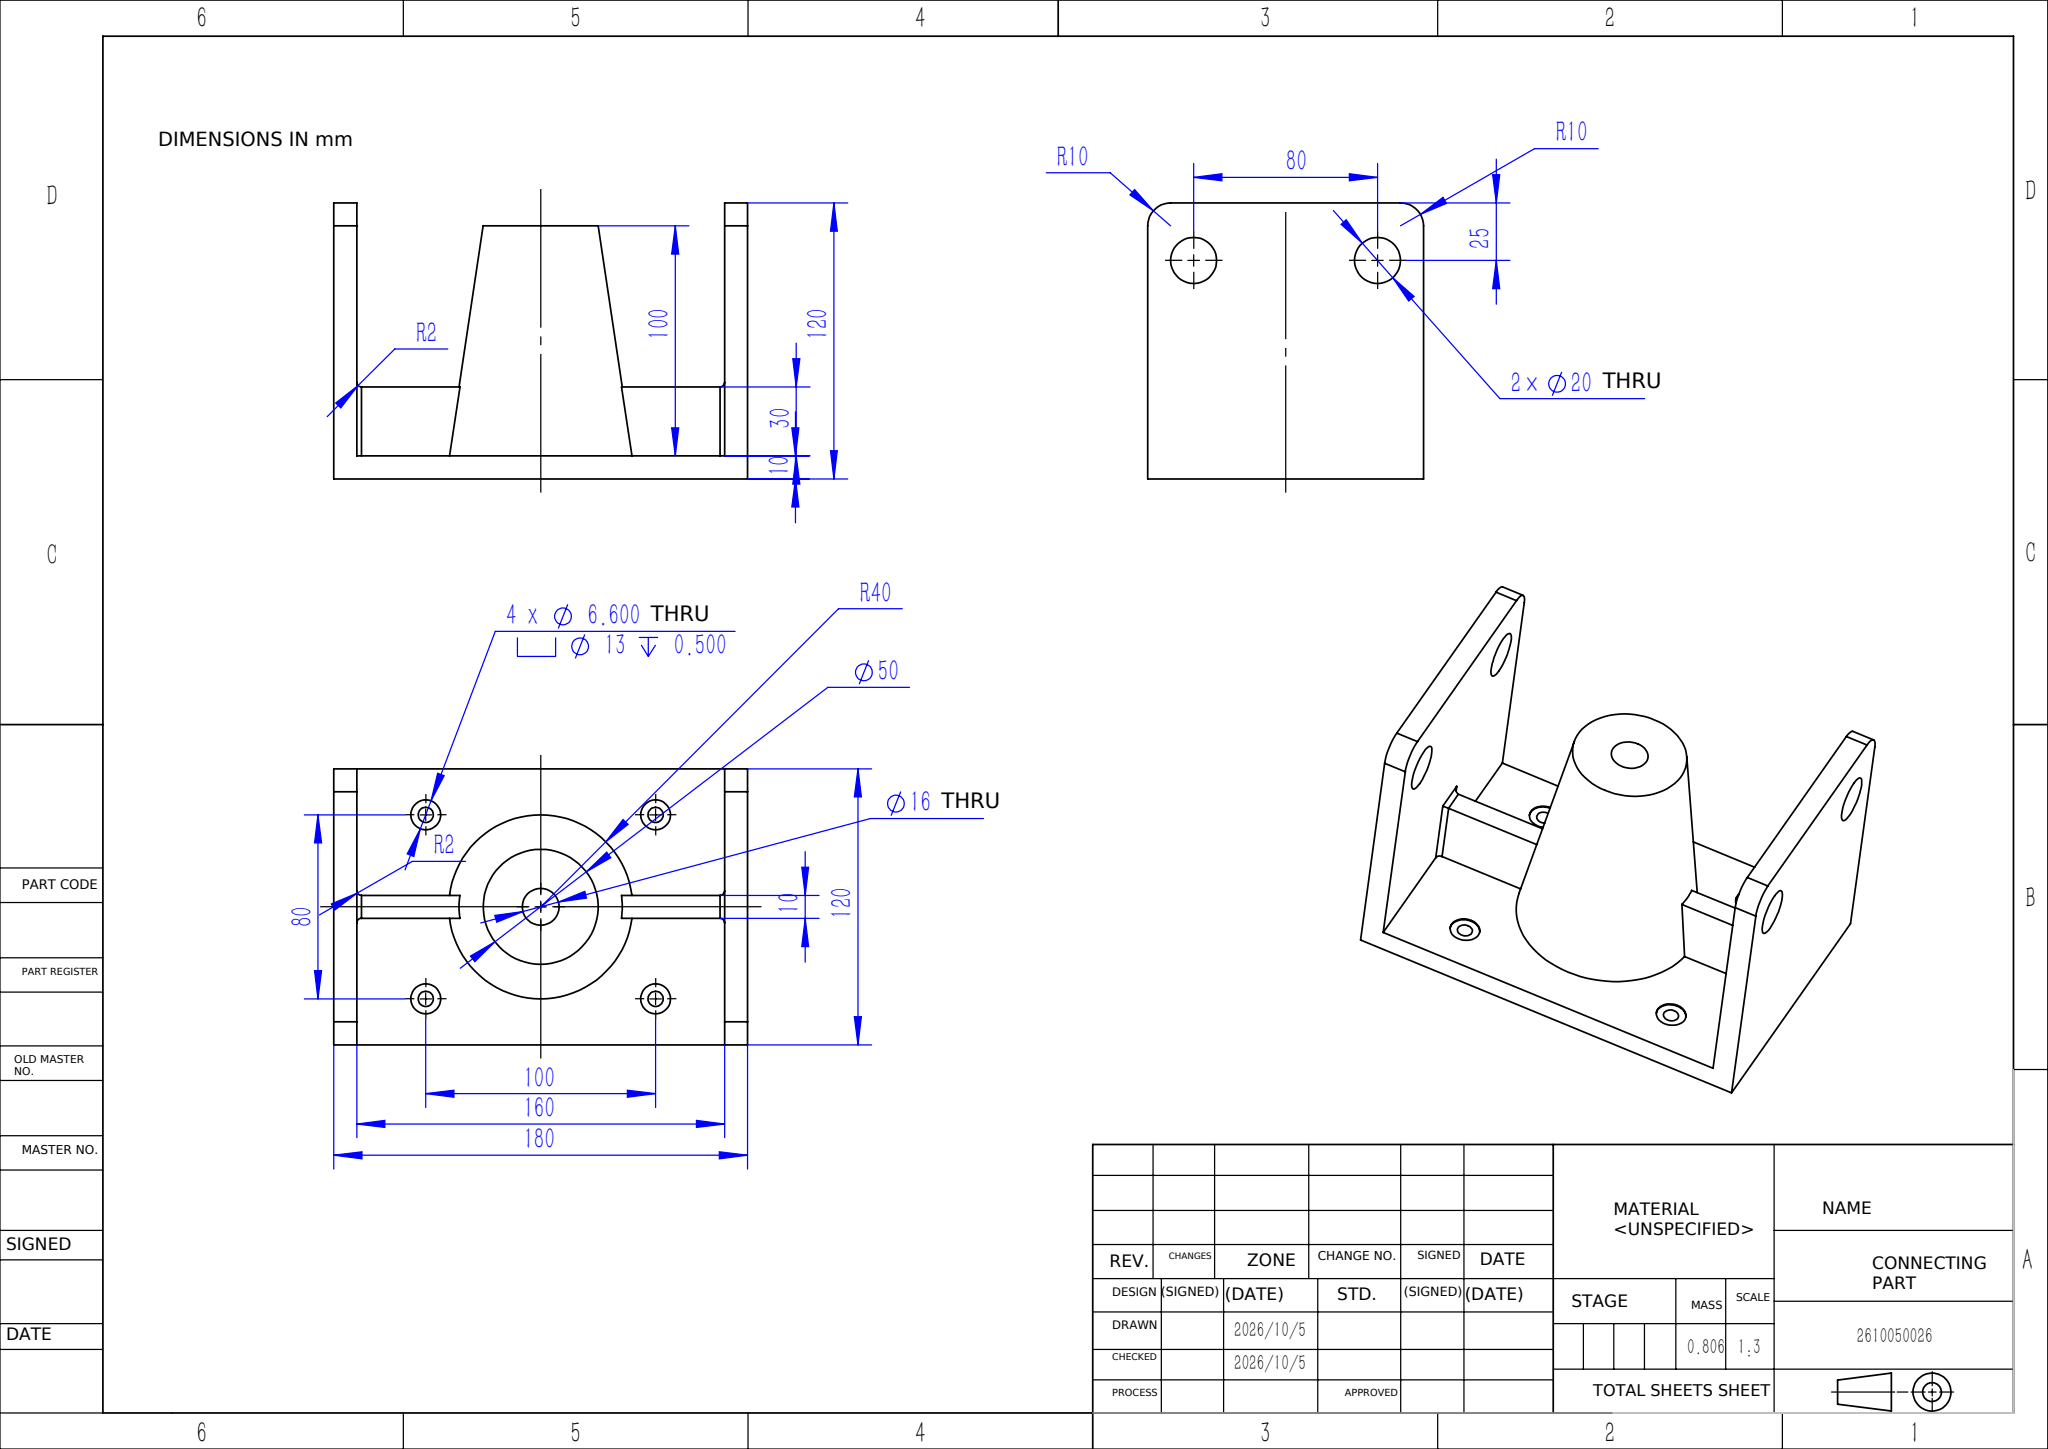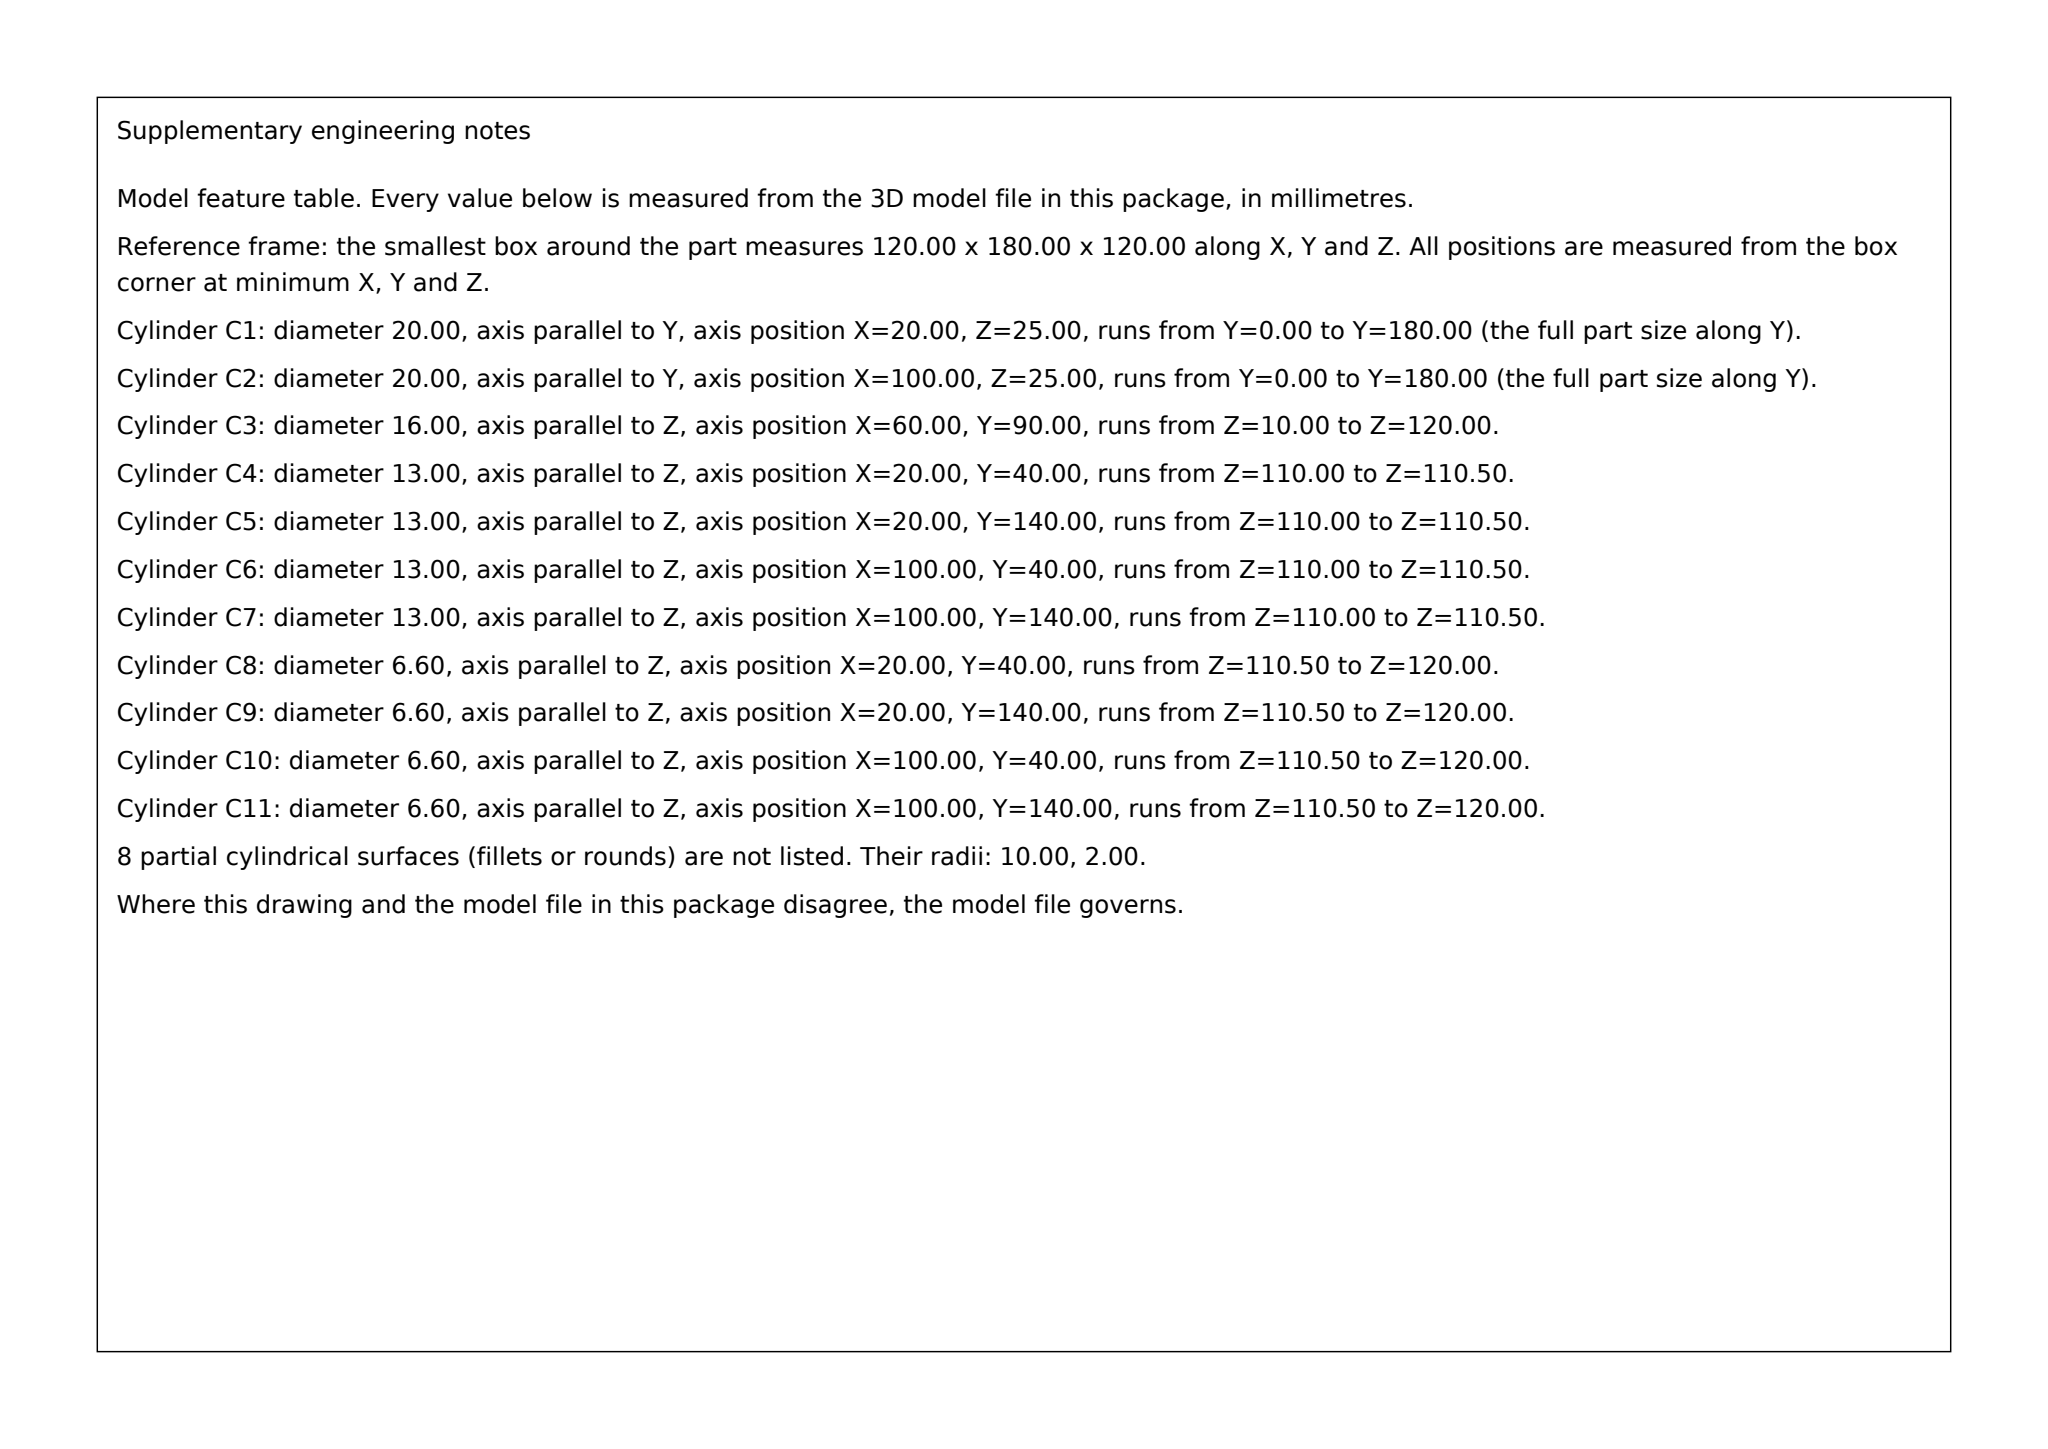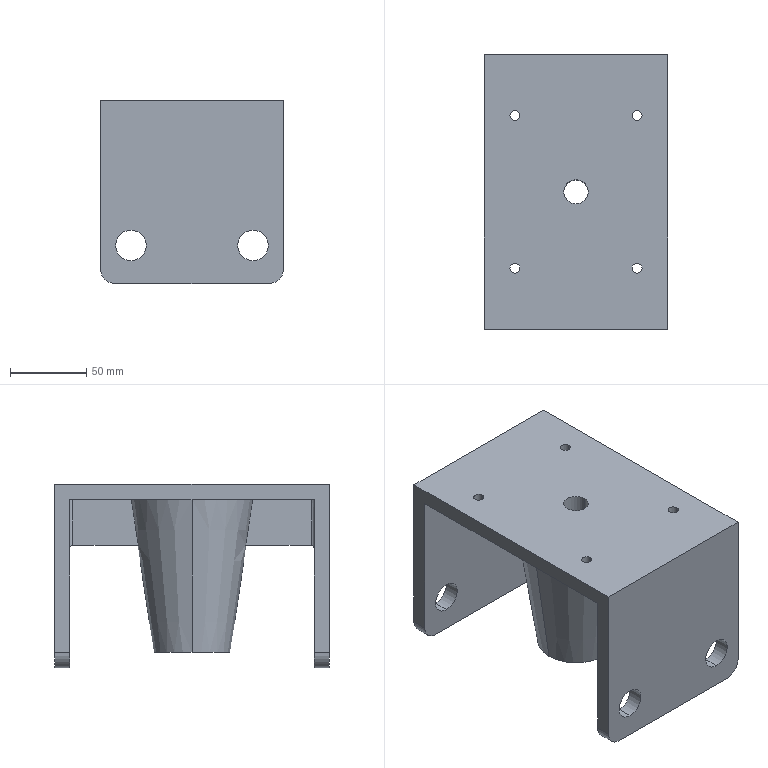Part | SolidWorks | mm | 1 solid | 60 faces | box 120 x 180 x 120 mm | volume 806154 mm3 | cylinder 36 | plane 22 | cone 2 | commonest cylinder face diameters 20 x12 13 x8 6.6 x8 4 x6 16 x2